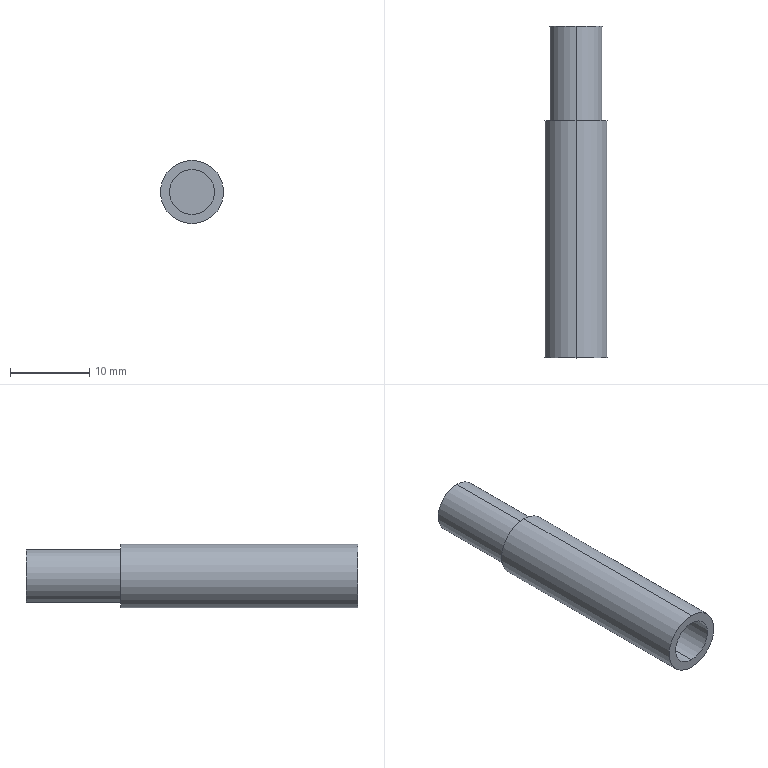Component | SolidWorks | NeedleSleeve-1 | 1 solid | 10 faces | box 8 x 42 x 8 mm | volume 885 mm3 | cylinder 6 | plane 4 | commonest cylinder face diameters 6.7 x2 8 x2 5.7 x2
build123d program:
from build123d import *

# Parameters (mm, degrees)
SKETCH1_R           = 4
SKETCH1_R_2         = 2.85
BOSS_EXTRUDE1_DEPTH = 30
SKETCH2_R           = 3.35
SKETCH2_R_2         = 2.85
BOSS_EXTRUDE2_DEPTH = 12
BOSS_EXTRUDE3_START = -1
SKETCH3_R           = 3.35
BOSS_EXTRUDE3_DEPTH = 1


with BuildPart() as part:
    # Sketch1 → Boss-Extrude1 (new body)
    with BuildSketch(Plane(origin=(0, 0, 0), x_dir=(1, 0, 0), z_dir=(0, 1, 0))):
        with Locations(Location((0, 0, 0), (0, 0, 270))):
            Circle(SKETCH1_R)
        with Locations(Location((0, 0, 0), (0, 0, 270))):
            Circle(SKETCH1_R_2, mode=Mode.SUBTRACT)
    extrude(amount=BOSS_EXTRUDE1_DEPTH)

    # Sketch2 → Boss-Extrude2 (add)
    with BuildSketch(Plane(origin=(0, 30, 0), x_dir=(1, 0, 0), z_dir=(0, 1, 0))):
        with Locations(Location((0, 0, 0), (0, 0, 270))):
            Circle(SKETCH2_R)
        with Locations(Location((0, 0, 0), (0, 0, 270))):
            Circle(SKETCH2_R_2, mode=Mode.SUBTRACT)
    extrude(amount=BOSS_EXTRUDE2_DEPTH)

    # Sketch3 → Boss-Extrude3 (add)
    with BuildSketch(Plane(origin=(0, 42, 0), x_dir=(1, 0, 0), z_dir=(0, 1, 0)).offset(BOSS_EXTRUDE3_START)):
        with Locations(Location((0, 0, 0), (0, 0, 270))):
            Circle(SKETCH3_R)
    extrude(amount=BOSS_EXTRUDE3_DEPTH)


solid = part.part

# Placed as in the assembly
solid = solid.moved(Location((431.234, 1432, -1930.507), (0, 0, 0)))
STEP:
#1=COLOUR_RGB('',0.7922,0.8196,0.9333);
#2=FILL_AREA_STYLE_COLOUR('',#1);
#3=FILL_AREA_STYLE('',(#2));
#4=SURFACE_STYLE_FILL_AREA(#3);
#5=SURFACE_SIDE_STYLE('',(#4));
#6=SURFACE_STYLE_USAGE(.BOTH.,#5);
#7=PRESENTATION_STYLE_ASSIGNMENT((#6));
#8=CARTESIAN_POINT('',(16.978,58.031,-75.872));
#9=VERTEX_POINT('',#8);
#10=CARTESIAN_POINT('',(16.978,58.031,-76.136));
#11=VERTEX_POINT('',#10);
#12=CARTESIAN_POINT('',(16.978,58.031,-76.004));
#13=DIRECTION('',(0.,1.,0.));
#14=DIRECTION('',(0.,0.,1.));
#15=AXIS2_PLACEMENT_3D('',#12,#13,#14);
#16=CIRCLE('',#15,0.1319);
#17=EDGE_CURVE('',#9,#11,#16,.T.);
#18=ORIENTED_EDGE('',*,*,#17,.F.);
#19=CARTESIAN_POINT('',(16.978,57.559,-75.872));
#20=VERTEX_POINT('',#19);
#21=CARTESIAN_POINT('',(16.978,58.031,-75.872));
#22=DIRECTION('',(0.,-1.,0.));
#23=VECTOR('',#22,39.37);
#24=LINE('',#21,#23);
#25=EDGE_CURVE('',#9,#20,#24,.T.);
#26=ORIENTED_EDGE('',*,*,#25,.T.);
#27=CARTESIAN_POINT('',(16.978,57.559,-76.136));
#28=VERTEX_POINT('',#27);
#29=CARTESIAN_POINT('',(16.978,57.559,-76.004));
#30=DIRECTION('',(0.,1.,0.));
#31=DIRECTION('',(0.,0.,1.));
#32=AXIS2_PLACEMENT_3D('',#29,#30,#31);
#33=CIRCLE('',#32,0.1319);
#34=EDGE_CURVE('',#20,#28,#33,.T.);
#35=ORIENTED_EDGE('',*,*,#34,.T.);
#36=CARTESIAN_POINT('',(16.978,58.031,-76.136));
#37=DIRECTION('',(0.,-1.,0.));
#38=VECTOR('',#37,39.37);
#39=LINE('',#36,#38);
#40=EDGE_CURVE('',#11,#28,#39,.T.);
#41=ORIENTED_EDGE('',*,*,#40,.F.);
#42=EDGE_LOOP('',(#18,#26,#35,#41));
#43=FACE_OUTER_BOUND('',#42,.T.);
#44=CARTESIAN_POINT('',(16.978,58.031,-76.004));
#45=DIRECTION('',(0.,-1.,0.));
#46=DIRECTION('',(0.,0.,-1.));
#47=AXIS2_PLACEMENT_3D('',#44,#45,#46);
#48=CYLINDRICAL_SURFACE('',#47,0.1319);
#49=ADVANCED_FACE('',(#43),#48,.T.);
#50=CARTESIAN_POINT('',(16.978,57.559,-75.847));
#51=VERTEX_POINT('',#50);
#52=CARTESIAN_POINT('',(16.978,57.559,-76.162));
#53=VERTEX_POINT('',#52);
#54=CARTESIAN_POINT('',(16.978,57.559,-76.004));
#55=DIRECTION('',(0.,1.,0.));
#56=DIRECTION('',(0.,0.,1.));
#57=AXIS2_PLACEMENT_3D('',#54,#55,#56);
#58=CIRCLE('',#57,0.1575);
#59=EDGE_CURVE('',#51,#53,#58,.T.);
#60=ORIENTED_EDGE('',*,*,#59,.F.);
#61=CARTESIAN_POINT('',(16.978,56.378,-75.847));
#62=VERTEX_POINT('',#61);
#63=CARTESIAN_POINT('',(16.978,57.559,-75.847));
#64=DIRECTION('',(0.,-1.,0.));
#65=VECTOR('',#64,39.37);
#66=LINE('',#63,#65);
#67=EDGE_CURVE('',#51,#62,#66,.T.);
#68=ORIENTED_EDGE('',*,*,#67,.T.);
#69=CARTESIAN_POINT('',(16.978,56.378,-76.162));
#70=VERTEX_POINT('',#69);
#71=CARTESIAN_POINT('',(16.978,56.378,-76.004));
#72=DIRECTION('',(0.,1.,0.));
#73=DIRECTION('',(0.,0.,1.));
#74=AXIS2_PLACEMENT_3D('',#71,#72,#73);
#75=CIRCLE('',#74,0.1575);
#76=EDGE_CURVE('',#62,#70,#75,.T.);
#77=ORIENTED_EDGE('',*,*,#76,.T.);
#78=CARTESIAN_POINT('',(16.978,57.559,-76.162));
#79=DIRECTION('',(0.,-1.,0.));
#80=VECTOR('',#79,39.37);
#81=LINE('',#78,#80);
#82=EDGE_CURVE('',#53,#70,#81,.T.);
#83=ORIENTED_EDGE('',*,*,#82,.F.);
#84=EDGE_LOOP('',(#60,#68,#77,#83));
#85=FACE_OUTER_BOUND('',#84,.T.);
#86=CARTESIAN_POINT('',(16.978,57.559,-76.004));
#87=DIRECTION('',(0.,-1.,0.));
#88=DIRECTION('',(0.,0.,-1.));
#89=AXIS2_PLACEMENT_3D('',#86,#87,#88);
#90=CYLINDRICAL_SURFACE('',#89,0.1575);
#91=ADVANCED_FACE('',(#85),#90,.T.);
#92=CARTESIAN_POINT('',(16.978,57.992,-76.116));
#93=VERTEX_POINT('',#92);
#94=CARTESIAN_POINT('',(16.978,57.992,-75.892));
#95=VERTEX_POINT('',#94);
#96=CARTESIAN_POINT('',(16.978,57.992,-76.004));
#97=DIRECTION('',(0.,1.,0.));
#98=DIRECTION('',(0.,0.,1.));
#99=AXIS2_PLACEMENT_3D('',#96,#97,#98);
#100=CIRCLE('',#99,0.1122);
#101=EDGE_CURVE('',#93,#95,#100,.T.);
#102=ORIENTED_EDGE('',*,*,#101,.T.);
#103=CARTESIAN_POINT('',(16.978,56.378,-75.892));
#104=VERTEX_POINT('',#103);
#105=CARTESIAN_POINT('',(16.978,57.559,-75.892));
#106=DIRECTION('',(0.,-1.,0.));
#107=VECTOR('',#106,39.37);
#108=LINE('',#105,#107);
#109=EDGE_CURVE('',#95,#104,#108,.T.);
#110=ORIENTED_EDGE('',*,*,#109,.T.);
#111=CARTESIAN_POINT('',(16.978,56.378,-76.116));
#112=VERTEX_POINT('',#111);
#113=CARTESIAN_POINT('',(16.978,56.378,-76.004));
#114=DIRECTION('',(0.,1.,0.));
#115=DIRECTION('',(0.,0.,1.));
#116=AXIS2_PLACEMENT_3D('',#113,#114,#115);
#117=CIRCLE('',#116,0.1122);
#118=EDGE_CURVE('',#112,#104,#117,.T.);
#119=ORIENTED_EDGE('',*,*,#118,.F.);
#120=CARTESIAN_POINT('',(16.978,57.559,-76.116));
#121=DIRECTION('',(0.,-1.,0.));
#122=VECTOR('',#121,39.37);
#123=LINE('',#120,#122);
#124=EDGE_CURVE('',#93,#112,#123,.T.);
#125=ORIENTED_EDGE('',*,*,#124,.F.);
#126=EDGE_LOOP('',(#102,#110,#119,#125));
#127=FACE_OUTER_BOUND('',#126,.T.);
#128=CARTESIAN_POINT('',(16.978,57.559,-76.004));
#129=DIRECTION('',(0.,-1.,0.));
#130=DIRECTION('',(0.,0.,-1.));
#131=AXIS2_PLACEMENT_3D('',#128,#129,#130);
#132=CYLINDRICAL_SURFACE('',#131,0.1122);
#133=ADVANCED_FACE('',(#127),#132,.F.);
#134=ORIENTED_EDGE('',*,*,#109,.F.);
#135=CARTESIAN_POINT('',(16.978,57.992,-76.004));
#136=DIRECTION('',(0.,1.,0.));
#137=DIRECTION('',(0.,0.,1.));
#138=AXIS2_PLACEMENT_3D('',#135,#136,#137);
#139=CIRCLE('',#138,0.1122);
#140=EDGE_CURVE('',#95,#93,#139,.T.);
#141=ORIENTED_EDGE('',*,*,#140,.T.);
#142=ORIENTED_EDGE('',*,*,#124,.T.);
#143=CARTESIAN_POINT('',(16.978,56.378,-76.004));
#144=DIRECTION('',(0.,1.,0.));
#145=DIRECTION('',(0.,0.,1.));
#146=AXIS2_PLACEMENT_3D('',#143,#144,#145);
#147=CIRCLE('',#146,0.1122);
#148=EDGE_CURVE('',#104,#112,#147,.T.);
#149=ORIENTED_EDGE('',*,*,#148,.F.);
#150=EDGE_LOOP('',(#134,#141,#142,#149));
#151=FACE_OUTER_BOUND('',#150,.T.);
#152=CARTESIAN_POINT('',(16.978,57.559,-76.004));
#153=DIRECTION('',(0.,-1.,0.));
#154=DIRECTION('',(0.,0.,-1.));
#155=AXIS2_PLACEMENT_3D('',#152,#153,#154);
#156=CYLINDRICAL_SURFACE('',#155,0.1122);
#157=ADVANCED_FACE('',(#151),#156,.F.);
#158=CARTESIAN_POINT('',(16.978,57.559,-76.004));
#159=DIRECTION('',(0.,1.,0.));
#160=DIRECTION('',(0.,0.,1.));
#161=AXIS2_PLACEMENT_3D('',#158,#159,#160);
#162=CIRCLE('',#161,0.1575);
#163=EDGE_CURVE('',#53,#51,#162,.T.);
#164=ORIENTED_EDGE('',*,*,#163,.T.);
#165=ORIENTED_EDGE('',*,*,#59,.T.);
#166=EDGE_LOOP('',(#164,#165));
#167=FACE_OUTER_BOUND('',#166,.T.);
#168=CARTESIAN_POINT('',(16.978,57.559,-76.004));
#169=DIRECTION('',(0.,1.,0.));
#170=DIRECTION('',(0.,0.,1.));
#171=AXIS2_PLACEMENT_3D('',#168,#169,#170);
#172=CIRCLE('',#171,0.1319);
#173=EDGE_CURVE('',#28,#20,#172,.T.);
#174=ORIENTED_EDGE('',*,*,#173,.F.);
#175=ORIENTED_EDGE('',*,*,#34,.F.);
#176=EDGE_LOOP('',(#174,#175));
#177=FACE_BOUND('',#176,.T.);
#178=CARTESIAN_POINT('',(16.978,57.559,-76.004));
#179=DIRECTION('',(0.,1.,0.));
#180=DIRECTION('',(0.,0.,1.));
#181=AXIS2_PLACEMENT_3D('',#178,#179,#180);
#182=PLANE('',#181);
#183=ADVANCED_FACE('',(#167,#177),#182,.T.);
#184=CARTESIAN_POINT('',(16.978,56.378,-76.004));
#185=DIRECTION('',(0.,1.,0.));
#186=DIRECTION('',(0.,0.,1.));
#187=AXIS2_PLACEMENT_3D('',#184,#185,#186);
#188=CIRCLE('',#187,0.1575);
#189=EDGE_CURVE('',#70,#62,#188,.T.);
#190=ORIENTED_EDGE('',*,*,#189,.F.);
#191=ORIENTED_EDGE('',*,*,#76,.F.);
#192=EDGE_LOOP('',(#190,#191));
#193=FACE_OUTER_BOUND('',#192,.T.);
#194=ORIENTED_EDGE('',*,*,#118,.T.);
#195=ORIENTED_EDGE('',*,*,#148,.T.);
#196=EDGE_LOOP('',(#194,#195));
#197=FACE_BOUND('',#196,.T.);
#198=CARTESIAN_POINT('',(16.978,56.378,-76.004));
#199=DIRECTION('',(0.,1.,0.));
#200=DIRECTION('',(0.,0.,1.));
#201=AXIS2_PLACEMENT_3D('',#198,#199,#200);
#202=PLANE('',#201);
#203=ADVANCED_FACE('',(#193,#197),#202,.F.);
#204=ORIENTED_EDGE('',*,*,#67,.F.);
#205=ORIENTED_EDGE('',*,*,#163,.F.);
#206=ORIENTED_EDGE('',*,*,#82,.T.);
#207=ORIENTED_EDGE('',*,*,#189,.T.);
#208=EDGE_LOOP('',(#204,#205,#206,#207));
#209=FACE_OUTER_BOUND('',#208,.T.);
#210=CARTESIAN_POINT('',(16.978,57.559,-76.004));
#211=DIRECTION('',(0.,-1.,0.));
#212=DIRECTION('',(0.,0.,-1.));
#213=AXIS2_PLACEMENT_3D('',#210,#211,#212);
#214=CYLINDRICAL_SURFACE('',#213,0.1575);
#215=ADVANCED_FACE('',(#209),#214,.T.);
#216=CARTESIAN_POINT('',(16.978,58.031,-76.004));
#217=DIRECTION('',(0.,1.,0.));
#218=DIRECTION('',(0.,0.,1.));
#219=AXIS2_PLACEMENT_3D('',#216,#217,#218);
#220=CIRCLE('',#219,0.1319);
#221=EDGE_CURVE('',#11,#9,#220,.T.);
#222=ORIENTED_EDGE('',*,*,#221,.T.);
#223=ORIENTED_EDGE('',*,*,#17,.T.);
#224=EDGE_LOOP('',(#222,#223));
#225=FACE_OUTER_BOUND('',#224,.T.);
#226=CARTESIAN_POINT('',(16.978,58.031,-76.004));
#227=DIRECTION('',(0.,1.,0.));
#228=DIRECTION('',(0.,0.,1.));
#229=AXIS2_PLACEMENT_3D('',#226,#227,#228);
#230=PLANE('',#229);
#231=ADVANCED_FACE('',(#225),#230,.T.);
#232=ORIENTED_EDGE('',*,*,#25,.F.);
#233=ORIENTED_EDGE('',*,*,#221,.F.);
#234=ORIENTED_EDGE('',*,*,#40,.T.);
#235=ORIENTED_EDGE('',*,*,#173,.T.);
#236=EDGE_LOOP('',(#232,#233,#234,#235));
#237=FACE_OUTER_BOUND('',#236,.T.);
#238=CARTESIAN_POINT('',(16.978,58.031,-76.004));
#239=DIRECTION('',(0.,-1.,0.));
#240=DIRECTION('',(0.,0.,-1.));
#241=AXIS2_PLACEMENT_3D('',#238,#239,#240);
#242=CYLINDRICAL_SURFACE('',#241,0.1319);
#243=ADVANCED_FACE('',(#237),#242,.T.);
#244=ORIENTED_EDGE('',*,*,#101,.F.);
#245=ORIENTED_EDGE('',*,*,#140,.F.);
#246=EDGE_LOOP('',(#244,#245));
#247=FACE_OUTER_BOUND('',#246,.T.);
#248=CARTESIAN_POINT('',(16.978,57.992,-76.004));
#249=DIRECTION('',(0.,1.,0.));
#250=DIRECTION('',(0.,0.,1.));
#251=AXIS2_PLACEMENT_3D('',#248,#249,#250);
#252=PLANE('',#251);
#253=ADVANCED_FACE('',(#247),#252,.F.);
#254=CLOSED_SHELL('',(#49,#91,#133,#157,#183,#203,#215,#231,#243,#253));
#255=MANIFOLD_SOLID_BREP('',#254);
#256=STYLED_ITEM('',(#7),#255);
#257=PRESENTATION_LAYER_ASSIGNMENT('','',(#256));
#258=CARTESIAN_POINT('',(0.,0.,0.));
#259=DIRECTION('',(0.,0.,1.));
#260=DIRECTION('',(1.,0.,0.));
#261=AXIS2_PLACEMENT_3D('',#258,#259,#260);
#262=(LENGTH_UNIT()NAMED_UNIT(*)SI_UNIT($,.METRE.));
#263=LENGTH_MEASURE_WITH_UNIT(LENGTH_MEASURE(0.0254),#262);
#264=DIMENSIONAL_EXPONENTS(1.,0.,0.,0.,0.,0.,0.);
#265=(CONVERSION_BASED_UNIT('',#263)LENGTH_UNIT()NAMED_UNIT(#264));
#266=UNCERTAINTY_MEASURE_WITH_UNIT(LENGTH_MEASURE(0.00001),#265,'','');
#267=(NAMED_UNIT(*)PLANE_ANGLE_UNIT()SI_UNIT($,.RADIAN.));
#268=(NAMED_UNIT(*)SI_UNIT($,.STERADIAN.)SOLID_ANGLE_UNIT());
#269=(GEOMETRIC_REPRESENTATION_CONTEXT(3)GLOBAL_UNCERTAINTY_ASSIGNED_CONTEXT((#266))GLOBAL_UNIT_ASSIGNED_CONTEXT((#265,#267,#268))REPRESENTATION_CONTEXT('',''));
#270=ADVANCED_BREP_SHAPE_REPRESENTATION('',(#255,#261),#269);
#271=(LENGTH_UNIT()NAMED_UNIT(*)SI_UNIT($,.METRE.));
#272=LENGTH_MEASURE_WITH_UNIT(LENGTH_MEASURE(0.0254),#271);
#273=DIMENSIONAL_EXPONENTS(1.,0.,0.,0.,0.,0.,0.);
#274=(CONVERSION_BASED_UNIT('',#272)LENGTH_UNIT()NAMED_UNIT(#273));
#275=UNCERTAINTY_MEASURE_WITH_UNIT(LENGTH_MEASURE(0.00001),#274,'','');
#276=(NAMED_UNIT(*)PLANE_ANGLE_UNIT()SI_UNIT($,.RADIAN.));
#277=(NAMED_UNIT(*)SI_UNIT($,.STERADIAN.)SOLID_ANGLE_UNIT());
#278=(GEOMETRIC_REPRESENTATION_CONTEXT(3)GLOBAL_UNCERTAINTY_ASSIGNED_CONTEXT((#275))GLOBAL_UNIT_ASSIGNED_CONTEXT((#274,#276,#277))REPRESENTATION_CONTEXT('',''));
#279=MECHANICAL_DESIGN_GEOMETRIC_PRESENTATION_REPRESENTATION('',(#256),#278);